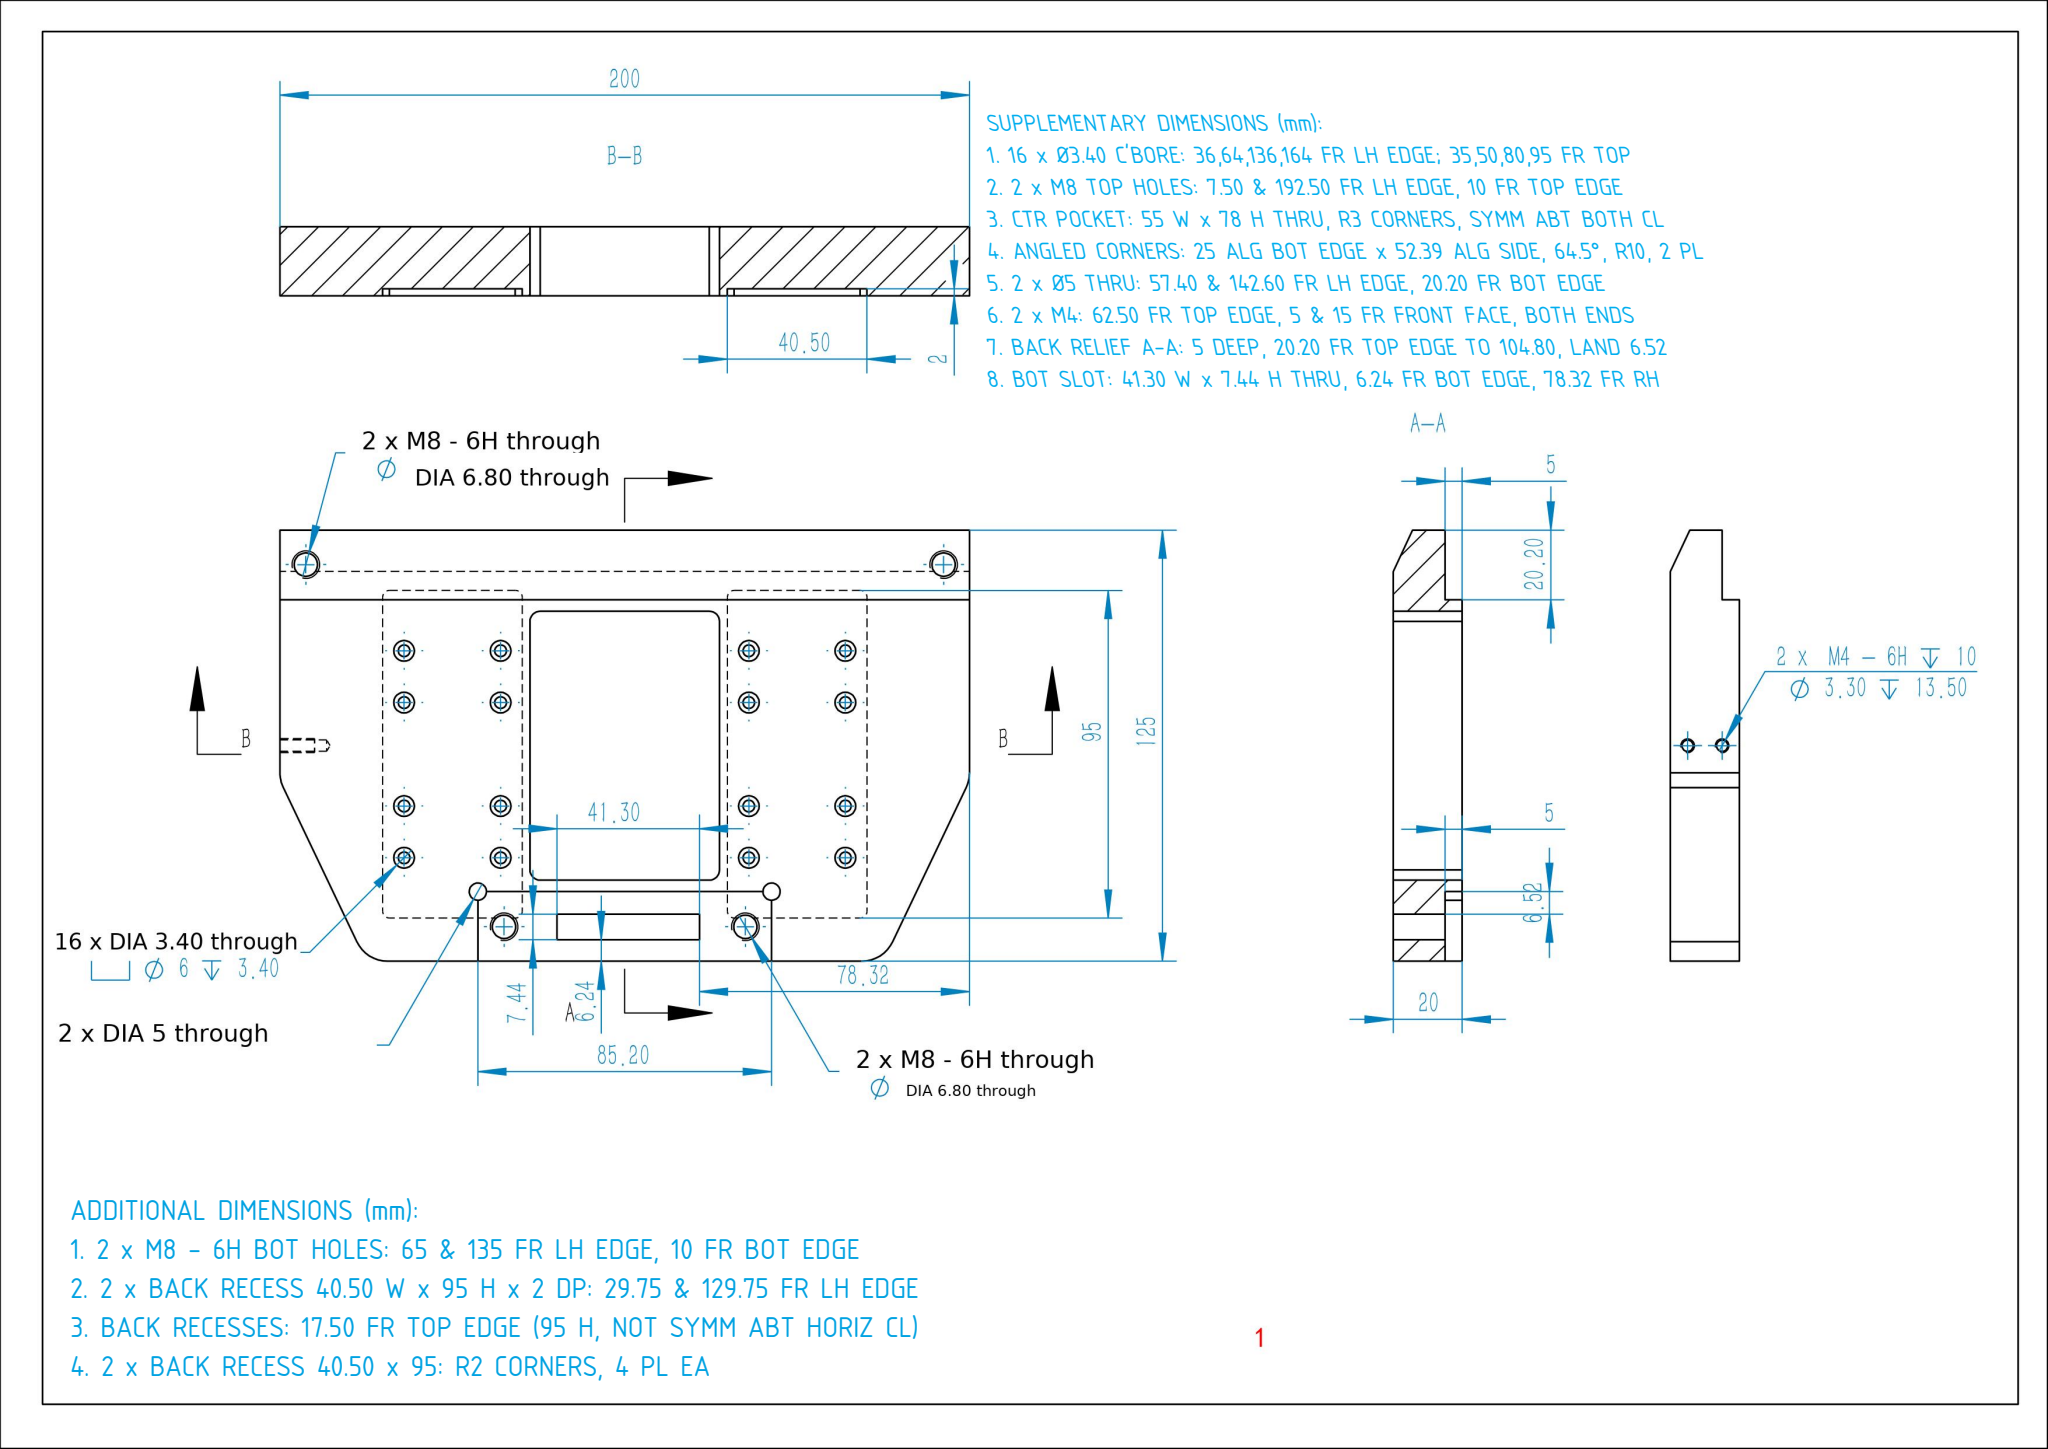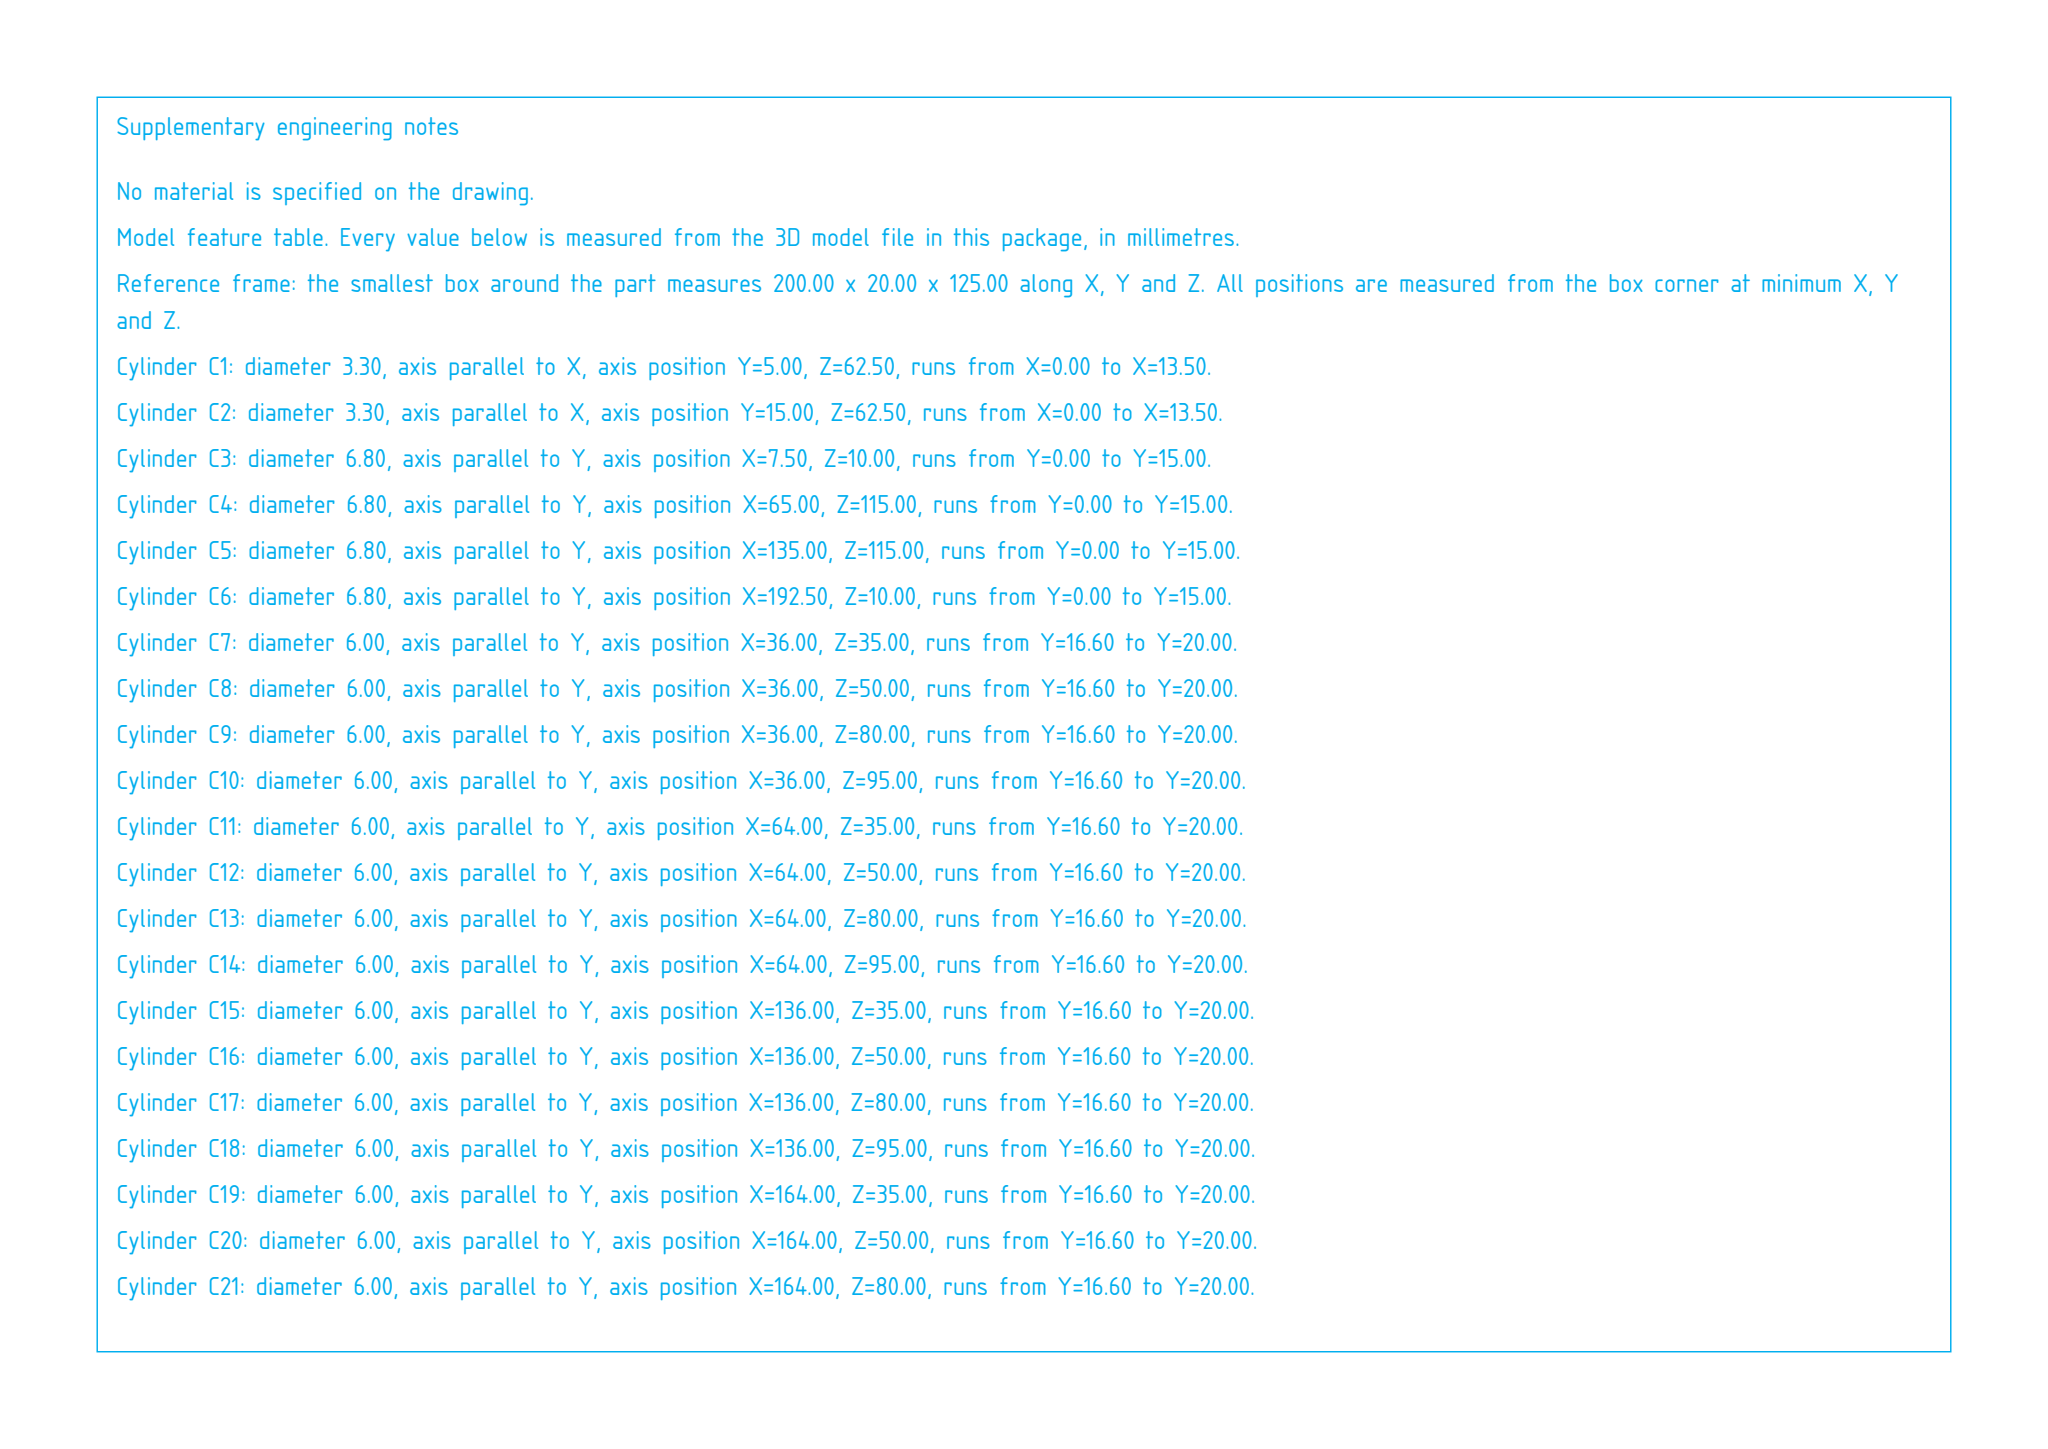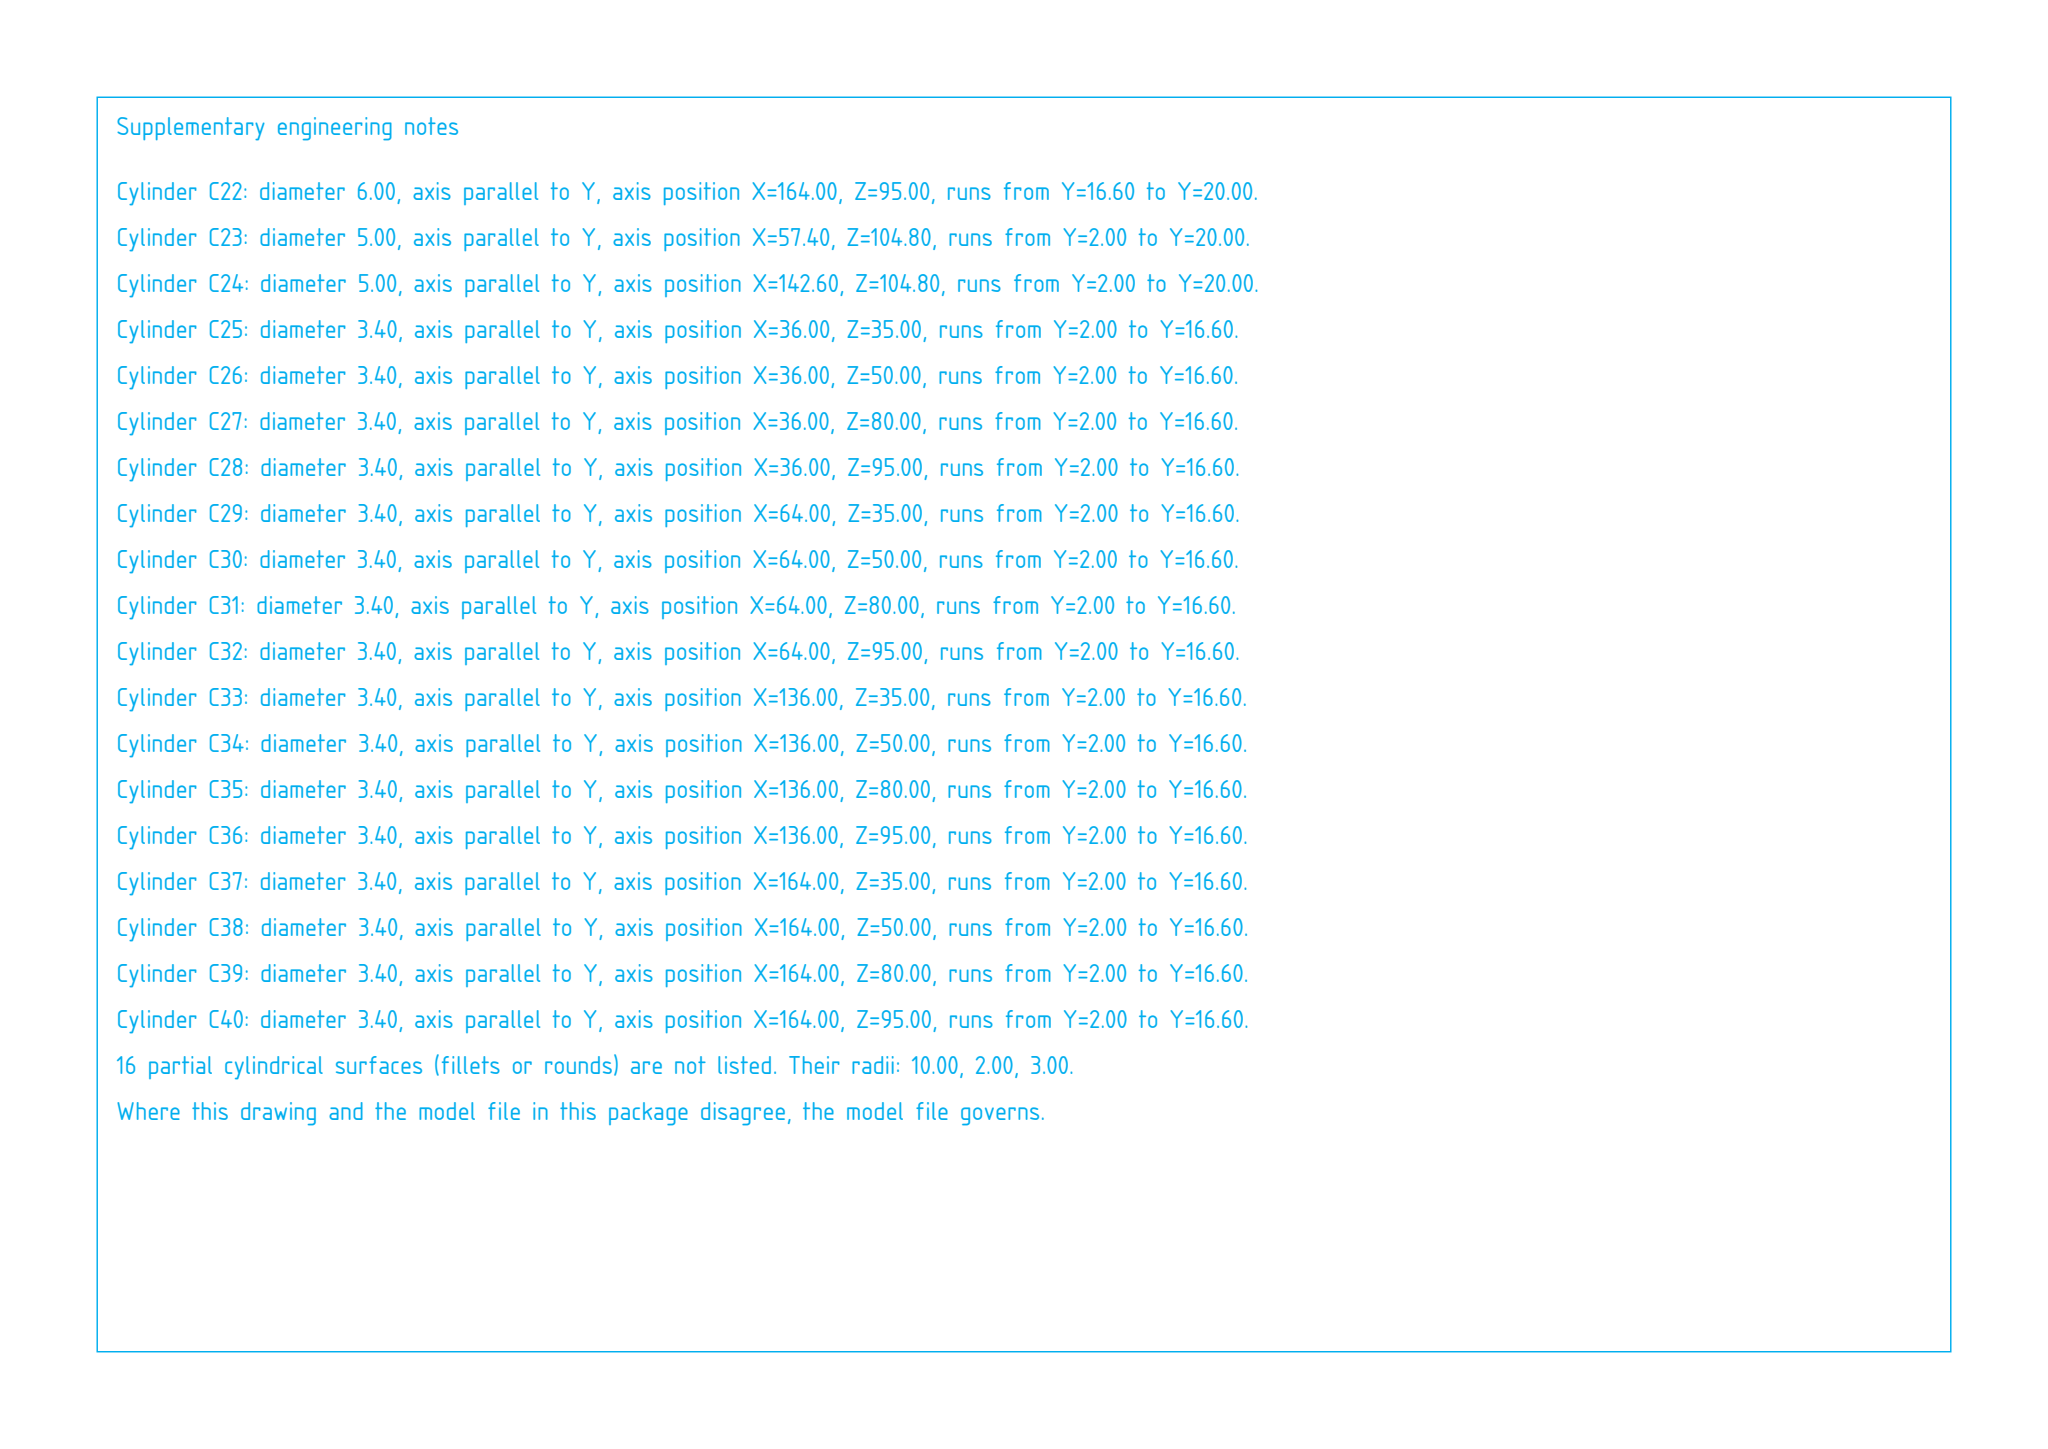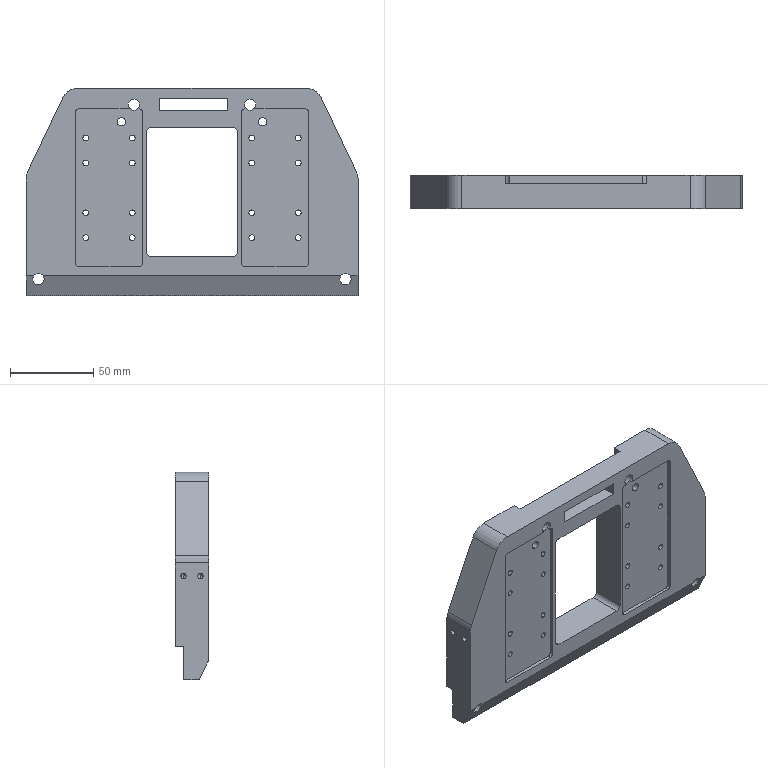Part | SolidWorks | mm | 1 solid | 151 faces | box 200 x 20 x 125 mm | volume 325712 mm3 | cylinder 96 | plane 51 | cone 4 | commonest cylinder face diameters 6 x36 3.4 x32 6.8 x8 4 x8 3.3 x4 5 x4 20 x4
build123d program:
from build123d import *

# Parameters (mm, degrees)
SKETCH1_W                                         = 200
SKETCH1_H                                         = 125
BOSS_EXTRUDE1_DEPTH                               = 10
SKETCH4_W                                         = 55
SKETCH4_H                                         = 78
CUT_EXTRUDE3_DEPTH                                = 120.609
FILLET1_R                                         = 3
CHAMFER1_SIZE                                     = 12
CHAMFER1_SIZE2                                    = 5.596
SKETCH5_W                                         = 20.2
SKETCH5_H                                         = 5
CUT_EXTRUDE4_DEPTH                                = 210.777
M8_TAPPED_HOLE1_D                                 = 6.8
SKETCH8_W                                         = 85.2
SKETCH8_H                                         = 40.4
CUT_EXTRUDE5_DEPTH                                = 5
F_5_0_5_DIAMETER_HOLE1_D                          = 5
CUT_EXTRUDE6_DEPTH                                = 120.609
FILLET2_R                                         = 10
M8_TAPPED_HOLE2_D                                 = 6.8
HOLE_SIZE_ACCORDING_TO_HEXAGON_SOCKET_D           = 3.4
HOLE_SIZE_ACCORDING_TO_HEXAGON_SOCKET_CBORE_D     = 6
HOLE_SIZE_ACCORDING_TO_HEXAGON_SOCKET_CBORE_DEPTH = 3.4
SKETCH16_W                                        = 40.5
SKETCH16_H                                        = 95
CUT_EXTRUDE7_DEPTH                                = 2
FILLET3_R                                         = 2
M4_TAPPED_HOLE1_D                                 = 3.3
M4_TAPPED_HOLE1_DEPTH                             = 13.5
M4_TAPPED_HOLE1_TIP                               = 0.9914
SKETCH19_W                                        = 41.305
SKETCH19_H                                        = 7.438
CUT_EXTRUDE8_DEPTH                                = 58


with BuildPart() as part:
    # Sketch1 → Boss-Extrude1 (new, symmetric)
    with BuildSketch(Plane(origin=(0, 0, 0), x_dir=(1, 0, 0), z_dir=(0, 1, 0))):
        Rectangle(SKETCH1_W, SKETCH1_H)
    extrude(amount=BOSS_EXTRUDE1_DEPTH, both=True)

    # Sketch4 → Cut-Extrude3 (cut, through all)
    with BuildSketch(Plane(origin=(0, 10, 0), x_dir=(1, 0, 0), z_dir=(0, 1, 0))):
        Rectangle(SKETCH4_W, SKETCH4_H)
    extrude(amount=-CUT_EXTRUDE3_DEPTH, mode=Mode.SUBTRACT)

    # Fillet1
    fillet1_edges = [part.edges().sort_by_distance(p)[0] for p in [
        (27.5, 0, -39),
        (27.5, 0, 39),
        (-27.5, 0, 39),
        (-27.5, 0, -39),
    ]]
    fillet(fillet1_edges, radius=FILLET1_R)

    # Chamfer1
    chamfer1_edges = [part.edges().sort_by_distance(p)[0] for p in [
        (0, -10, -62.5),
    ]]
    chamfer1_side = [part.faces().sort_by_distance(p)[0] for p in [
        (0, -10, 41.358),
    ]]
    chamfer(chamfer1_edges, length=CHAMFER1_SIZE, length2=CHAMFER1_SIZE2, reference=chamfer1_side[0])

    # Sketch5 → Cut-Extrude4 (cut, through all)
    with BuildSketch(Plane(origin=(100, 0, 0), x_dir=(0, 0, -1), z_dir=(1, 0, 0))):
        with Locations((52.4, 7.5)):
            Rectangle(SKETCH5_W, SKETCH5_H)
    extrude(amount=-CUT_EXTRUDE4_DEPTH, mode=Mode.SUBTRACT)

    # M8 Tapped Hole1 (through all)
    with Locations(Plane(origin=(0, 10, 0), x_dir=(1, 0, 0), z_dir=(0, 1, 0))):
        with Locations((-92.5, 52.5), (92.5, 52.5)):
            Hole(M8_TAPPED_HOLE1_D / 2)

    # Sketch8 → Cut-Extrude5 (cut)
    with BuildSketch(Plane(origin=(0, 10, 0), x_dir=(1, 0, 0), z_dir=(0, 1, 0))):
        with Locations((0, -62.5)):
            Rectangle(SKETCH8_W, SKETCH8_H)
    extrude(amount=-CUT_EXTRUDE5_DEPTH, mode=Mode.SUBTRACT)

    # 5.0 _5_ Diameter Hole1 (through all)
    with Locations(Plane(origin=(0, 10, 0), x_dir=(1, 0, 0), z_dir=(0, 1, 0))):
        with Locations((-42.6, -42.3), (42.6, -42.3)):
            Hole(F_5_0_5_DIAMETER_HOLE1_D / 2)

    # Sketch11 → Cut-Extrude6 (cut, through all)
    with BuildSketch(Plane(origin=(0, 10, 0), x_dir=(1, 0, 0), z_dir=(0, 1, 0))):
        Polygon((-100, -10.1), (-75, -62.5), (-100, -62.5), align=None)
    cut_extrude6 = extrude(amount=-CUT_EXTRUDE6_DEPTH, mode=Mode.SUBTRACT)

    # Mirror1: Cut-Extrude6 across plane
    add(cut_extrude6.mirror(Plane(origin=(0, 0, 0), x_dir=(0, 0, 1), z_dir=(1, 0, 0))), mode=Mode.SUBTRACT)

    # Fillet2
    fillet2_edges = [part.edges().sort_by_distance(p)[0] for p in [
        (-100, 0, 10.1),
        (-75, 0, 62.5),
        (100, 0, 10.1),
        (75, 0, 62.5),
    ]]
    fillet(fillet2_edges, radius=FILLET2_R)

    # M8 Tapped Hole2 (through all)
    with Locations(Plane(origin=(0, 5, 0), x_dir=(1, 0, 0), z_dir=(0, 1, 0))):
        with Locations((-35, -52.5), (35, -52.5)):
            Hole(M8_TAPPED_HOLE2_D / 2)

    # Hole Size _According to_ Hexagon Socket (through all)
    with Locations(Plane(origin=(0, 10, 0), x_dir=(1, 0, 0), z_dir=(0, 1, 0))):
        with Locations((-64, -32.5), (-36, -32.5), (-64, -17.5), (-36, -17.5), (-64, 12.5), (-36, 12.5), (-64, 27.5), (-36, 27.5), (36, -17.5), (64, -17.5), (36, -32.5), (64, -32.5), (36, 27.5), (64, 27.5), (36, 12.5), (64, 12.5)):
            CounterBoreHole(HOLE_SIZE_ACCORDING_TO_HEXAGON_SOCKET_D / 2, HOLE_SIZE_ACCORDING_TO_HEXAGON_SOCKET_CBORE_D / 2, HOLE_SIZE_ACCORDING_TO_HEXAGON_SOCKET_CBORE_DEPTH)

    # Sketch16 → Cut-Extrude7 (cut)
    with BuildSketch(Plane.XZ.offset(10)):
        with Locations((-50, 2.5)):
            Rectangle(SKETCH16_W, SKETCH16_H)
        with Locations((50, 2.5)):
            Rectangle(SKETCH16_W, SKETCH16_H)
    extrude(amount=-CUT_EXTRUDE7_DEPTH, mode=Mode.SUBTRACT)

    # Fillet3
    fillet3_edges = [part.edges().sort_by_distance(p)[0] for p in [
        (-70.25, -9, 50),
        (-29.75, -9, 50),
        (-29.75, -9, -45),
        (-70.25, -9, -45),
        (29.75, -9, 50),
        (70.25, -9, 50),
        (70.25, -9, -45),
        (29.75, -9, -45),
    ]]
    fillet(fillet3_edges, radius=FILLET3_R)

    # M4 Tapped Hole1
    with Locations(Plane.ZY.offset(100)):
        with Locations((0, 5), (0, -5)):
            Hole(M4_TAPPED_HOLE1_D / 2, depth=M4_TAPPED_HOLE1_DEPTH)
            with Locations((0, 0, -(M4_TAPPED_HOLE1_DEPTH + M4_TAPPED_HOLE1_TIP / 2))):  # 118° drill point
                Cone(0, M4_TAPPED_HOLE1_D / 2, M4_TAPPED_HOLE1_TIP, mode=Mode.SUBTRACT)

    # Sketch19 → Cut-Extrude8 (cut)
    with BuildSketch(Plane(origin=(0, 5, 0), x_dir=(1, 0, 0), z_dir=(0, 1, 0))):
        with Locations((1.029, -52.541)):
            Rectangle(SKETCH19_W, SKETCH19_H)
    extrude(amount=-CUT_EXTRUDE8_DEPTH, mode=Mode.SUBTRACT)


solid = part.part